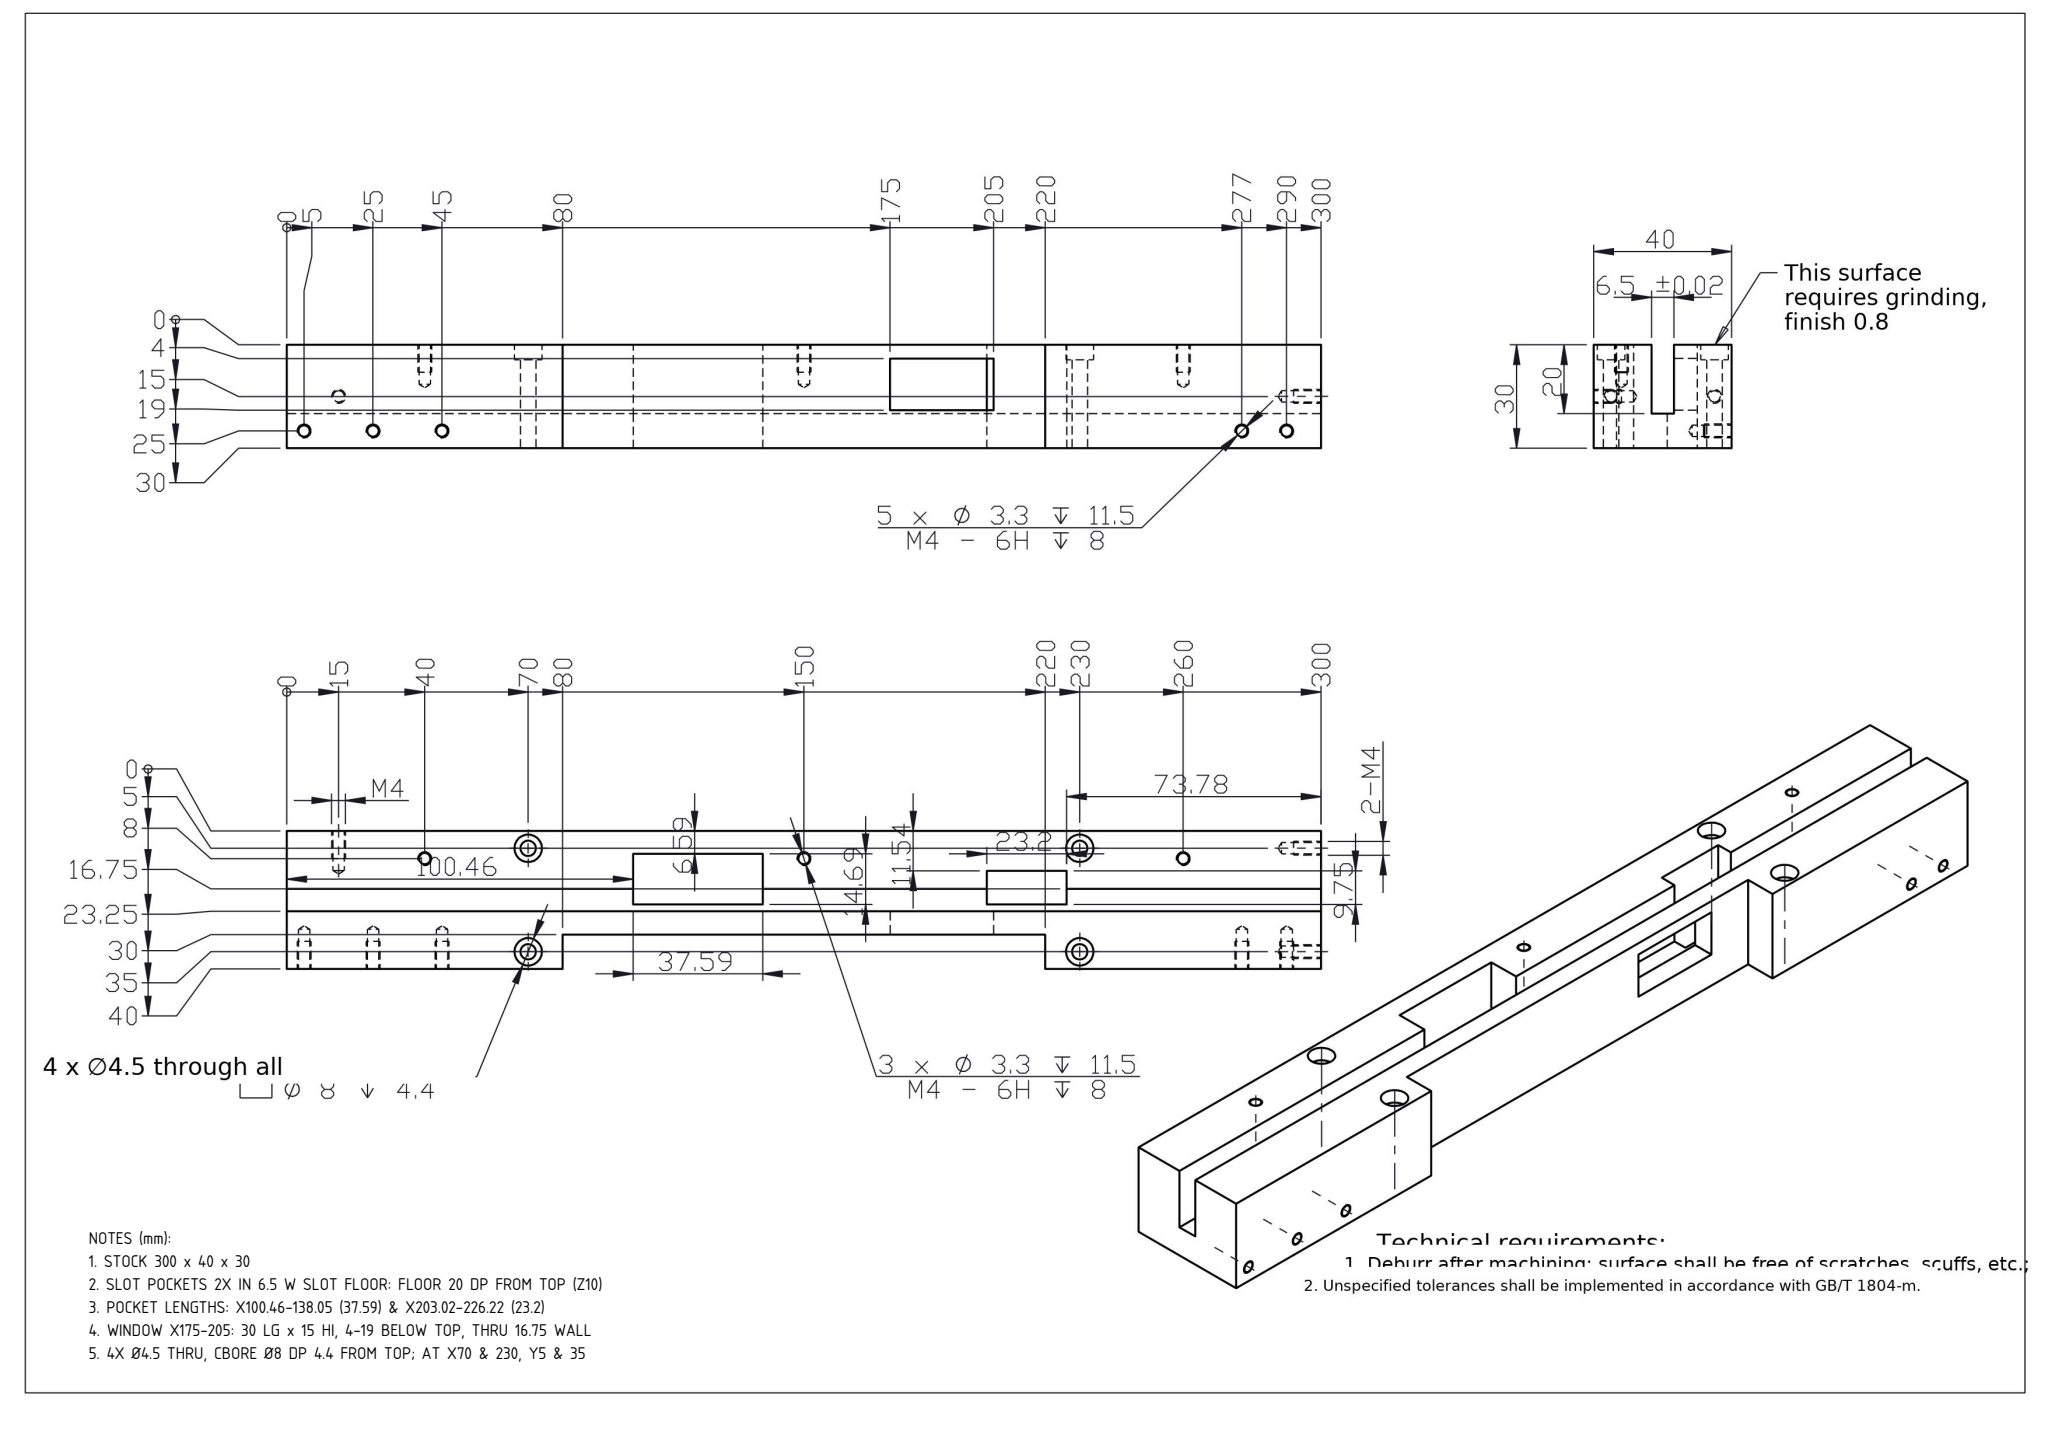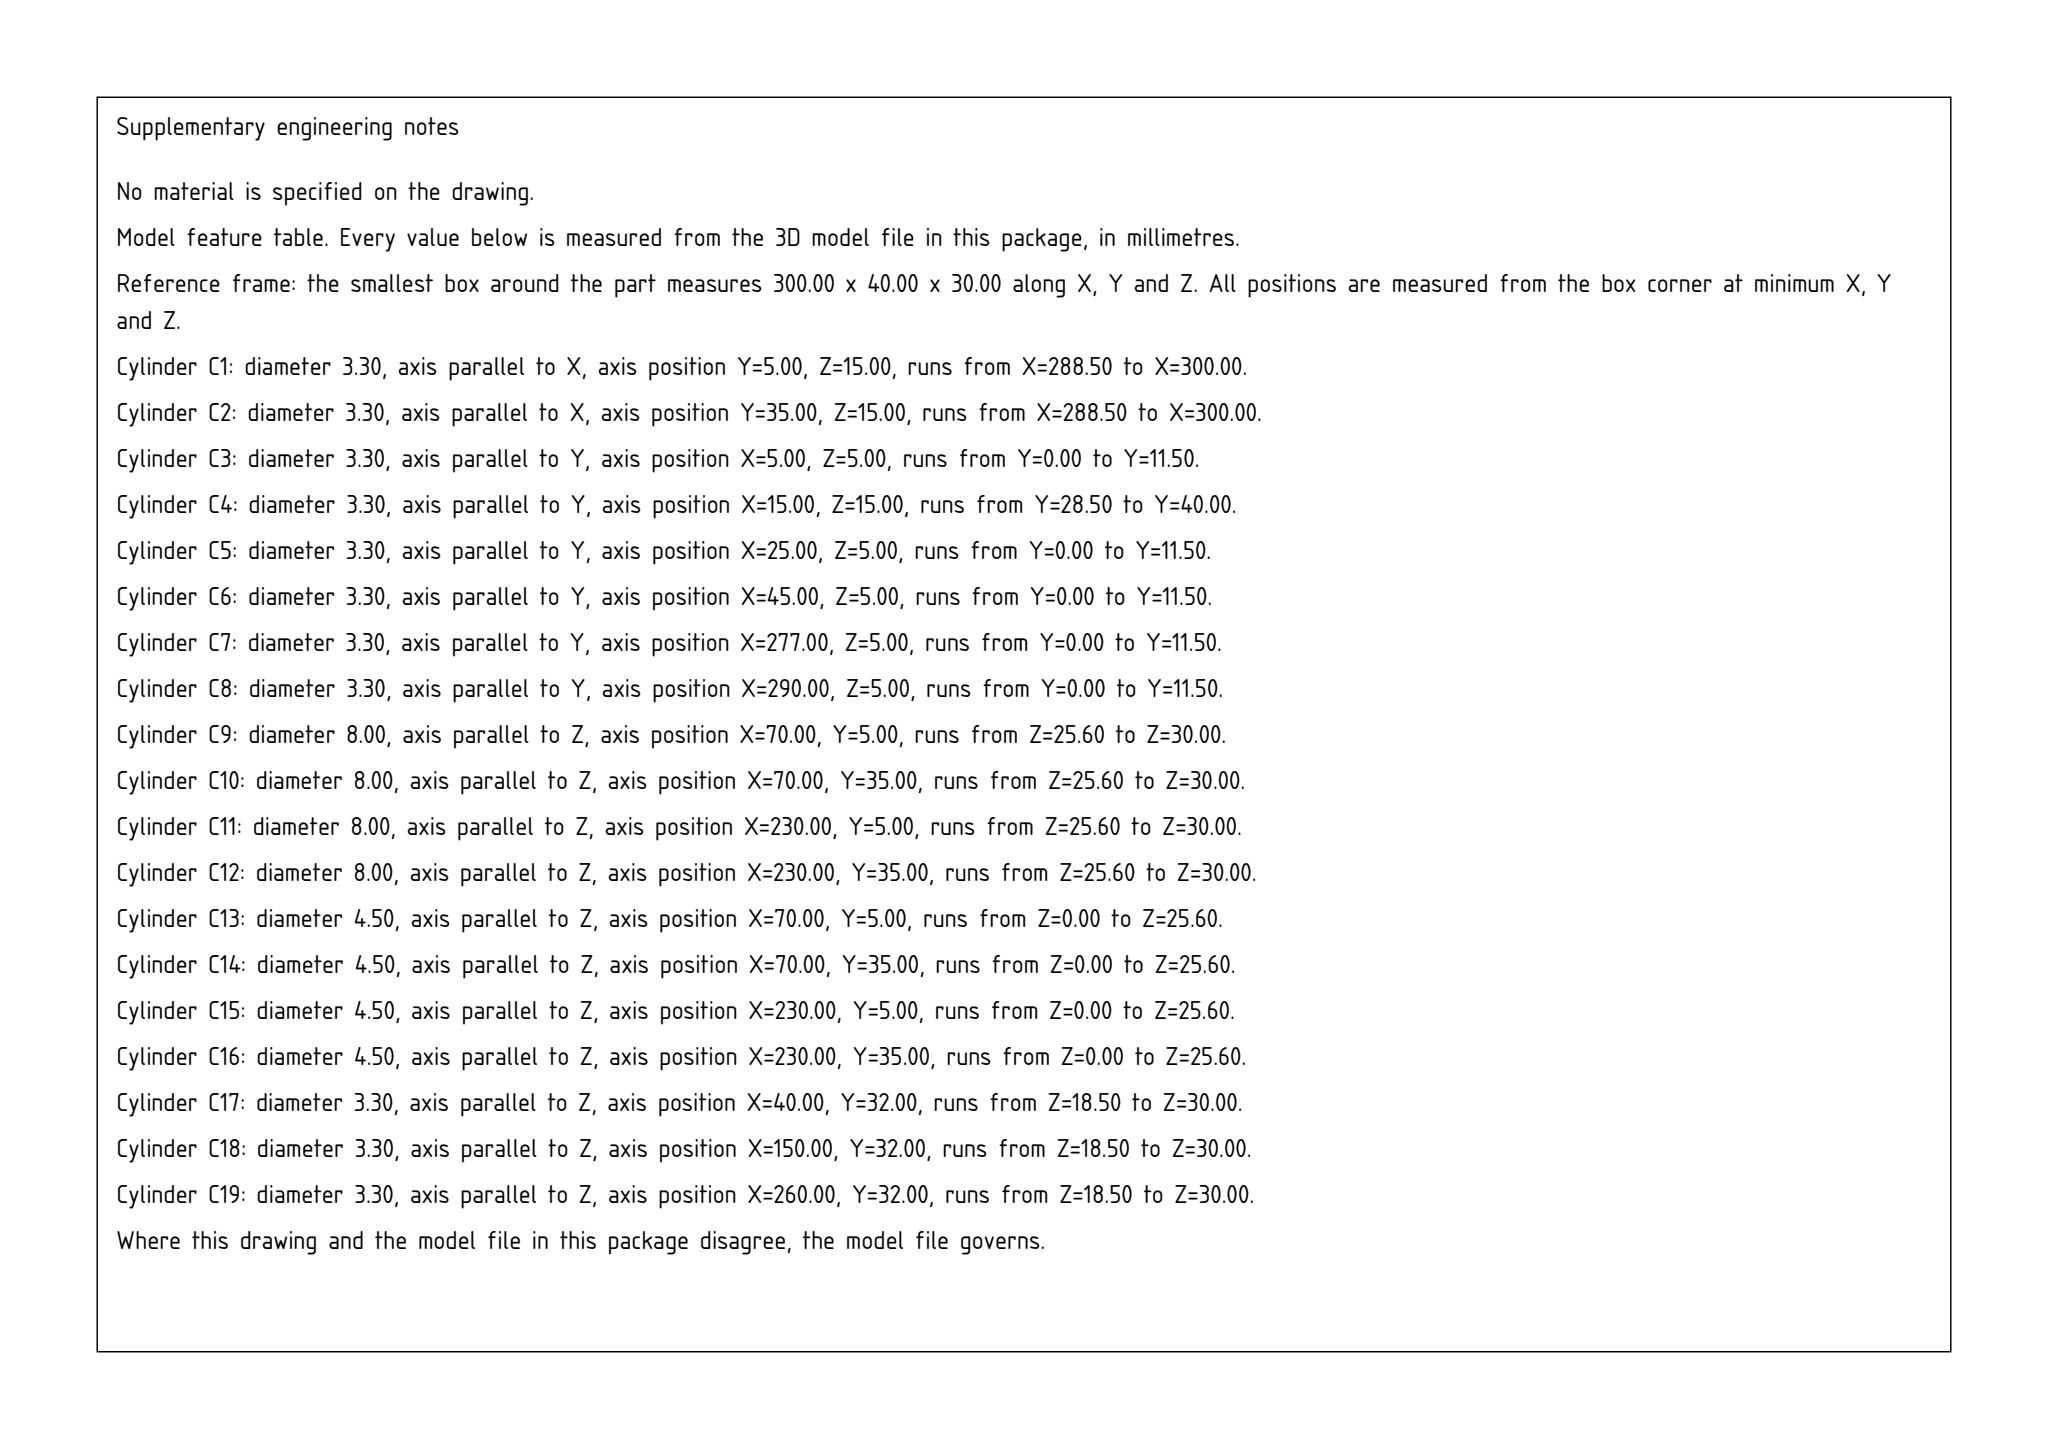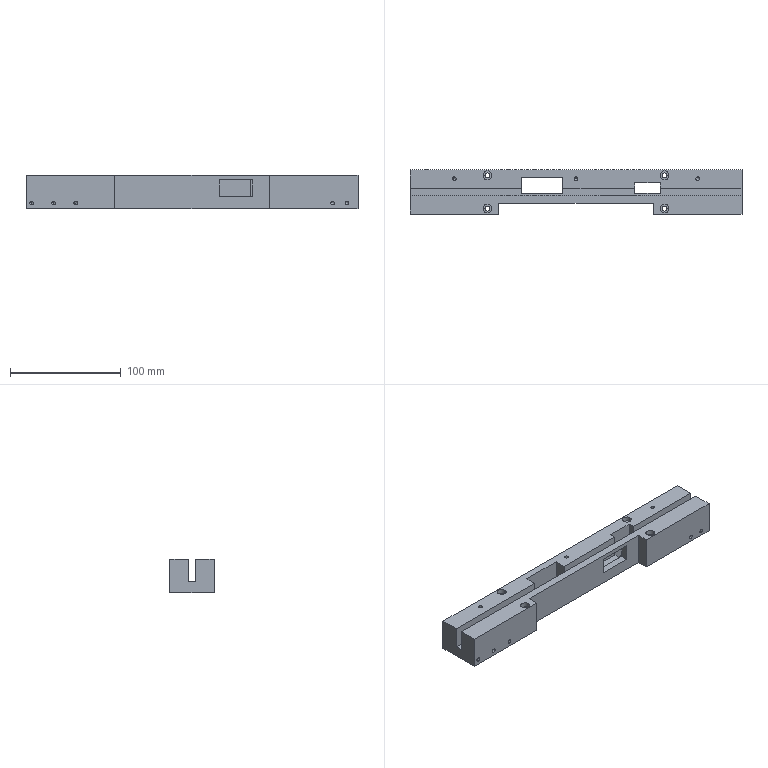Part | SolidWorks | mm | 1 solid | 92 faces | box 300 x 40 x 30 mm | volume 254494 mm3 | cylinder 38 | plane 32 | cone 22 | commonest cylinder face diameters 3.3 x22 8 x8 4.5 x8
Drawing notes:
STOCK 300 x 40 x 30 | from the solid: bbox_xyz 300.0 x 40.0 x 30.0
SLOT POCKETS 2X IN 6.5 W SLOT FLOOR: FLOOR 20 DP FROM TOP (Z10) | from the solid: y-planes 16.75 & 23.25 = 6.5 W; pocket floor z=10.0, 20 below z=30 top face
POCKET LENGTHS: X100.46-138.05 (37.59) & X203.02-226.22 (23.2) | from the solid: x-planes 100.46, 138.05, 203.02, 226.22
WINDOW X175-205: 30 LG x 15 HI, 4-19 BELOW TOP, THRU 16.75 WALL | from the solid: x-planes 175.0 & 205.0; z-planes 11.0 & 26.0; wall y=0 to y=16.75
4X Ø4.5 THRU, CBORE Ø8 DP 4.4 FROM TOP; AT X70 & 230, Y5 & 35 | from the solid: Ø4.5 axis z L25.6 and Ø8 axis z L4.4 at (70,5),(70,35),(230,5),(230,35); z-planes 25.6 & 30.0
build123d program:
from build123d import *

# Parameters (mm, degrees)
SKETCH1_W                                       = 300
SKETCH1_H                                       = 40
BOSS_EXTRUDE1_DEPTH                             = 30
SKETCH2_W                                       = 300
SKETCH2_H                                       = 6.5
CUT_EXTRUDE1_DEPTH                              = 20
M4_HEX_SOCKET_HEAD_CAP_SCREW_CBORE2_D           = 4.5
M4_HEX_SOCKET_HEAD_CAP_SCREW_CBORE2_CBORE_D     = 8
M4_HEX_SOCKET_HEAD_CAP_SCREW_CBORE2_CBORE_DEPTH = 4.4
M4_TAPPED_HOLE1_D                               = 3.3
M4_TAPPED_HOLE1_DEPTH                           = 11.5
M4_TAPPED_HOLE1_TIP                             = 0.9914
SKETCH13_W                                      = 140
SKETCH13_H                                      = 30
CUT_EXTRUDE2_DEPTH                              = 10
CUT_EXTRUDE3_REACH                              = 304.985
SKETCH14_W                                      = 30
SKETCH14_H                                      = 15
M4_TAPPED_HOLE2_D                               = 3.3
M4_TAPPED_HOLE2_DEPTH                           = 11.5
M4_TAPPED_HOLE2_TIP                             = 0.9914
M4_TAPPED_HOLE3_D                               = 3.3
M4_TAPPED_HOLE3_DEPTH                           = 11.5
M4_TAPPED_HOLE3_TIP                             = 0.9914
M4_TAPPED_HOLE4_D                               = 3.3
M4_TAPPED_HOLE4_DEPTH                           = 11.5
M4_TAPPED_HOLE4_TIP                             = 0.9914
M4_TAPPED_HOLE5_D                               = 3.3
M4_TAPPED_HOLE5_DEPTH                           = 11.5
M4_TAPPED_HOLE5_TIP                             = 0.9914
SKETCH23_W                                      = 23.203
SKETCH23_H                                      = 9.745
SKETCH23_W_2                                    = 37.588
SKETCH23_H_2                                    = 14.695
CUT_EXTRUDE4_DEPTH                              = 74


with BuildPart() as part:
    # Sketch1 → Boss-Extrude1 (new body)
    with BuildSketch(Plane.XY):
        with Locations((150, -20)):
            Rectangle(SKETCH1_W, SKETCH1_H)
    extrude(amount=BOSS_EXTRUDE1_DEPTH)

    # Sketch2 → Cut-Extrude1 (cut)
    with BuildSketch(Plane.XY.offset(30)):
        with Locations((150, -20)):
            Rectangle(SKETCH2_W, SKETCH2_H)
    extrude(amount=-CUT_EXTRUDE1_DEPTH, mode=Mode.SUBTRACT)

    # M4 Hex Socket Head Cap Screw CBORE2 (through all)
    with Locations(Plane.XY.offset(30)):
        with Locations((70, -35), (230, -35), (230, -5), (70, -5)):
            CounterBoreHole(M4_HEX_SOCKET_HEAD_CAP_SCREW_CBORE2_D / 2, M4_HEX_SOCKET_HEAD_CAP_SCREW_CBORE2_CBORE_D / 2, M4_HEX_SOCKET_HEAD_CAP_SCREW_CBORE2_CBORE_DEPTH)

    # M4 Tapped Hole1
    with Locations(Plane(origin=(0, -40, 0), x_dir=(-1, 0, 0), z_dir=(0, -1, 0))):
        with Locations((-25, -5), (-45, -5), (-5, -5)):
            Hole(M4_TAPPED_HOLE1_D / 2, depth=M4_TAPPED_HOLE1_DEPTH)
            with Locations((0, 0, -(M4_TAPPED_HOLE1_DEPTH + M4_TAPPED_HOLE1_TIP / 2))):  # 118° drill point
                Cone(0, M4_TAPPED_HOLE1_D / 2, M4_TAPPED_HOLE1_TIP, mode=Mode.SUBTRACT)

    # Sketch13 → Cut-Extrude2 (cut)
    with BuildSketch(Plane.XZ.offset(40)):
        with Locations((150, 15)):
            Rectangle(SKETCH13_W, SKETCH13_H)
    extrude(amount=-CUT_EXTRUDE2_DEPTH, mode=Mode.SUBTRACT)

    # Sketch14 → Cut-Extrude3 (cut, up to next)
    with BuildSketch(Plane.XZ.offset(30), mode=Mode.PRIVATE) as cut_extrude3_sk1:
        with Locations((190, 18.5)):
            Rectangle(SKETCH14_W, SKETCH14_H)
    cut_extrude3_tool1 = extrude(cut_extrude3_sk1.sketch, amount=-CUT_EXTRUDE3_REACH, mode=Mode.PRIVATE) & part.part
    add(cut_extrude3_tool1.solids().sort_by_distance((190, -30, 18.5))[0], mode=Mode.SUBTRACT)

    # M4 Tapped Hole2
    with Locations(Plane(origin=(0, -40, 0), x_dir=(-1, 0, 0), z_dir=(0, -1, 0))):
        with Locations((-290, -5), (-277, -5)):
            Hole(M4_TAPPED_HOLE2_D / 2, depth=M4_TAPPED_HOLE2_DEPTH)
            with Locations((0, 0, -(M4_TAPPED_HOLE2_DEPTH + M4_TAPPED_HOLE2_TIP / 2))):  # 118° drill point
                Cone(0, M4_TAPPED_HOLE2_D / 2, M4_TAPPED_HOLE2_TIP, mode=Mode.SUBTRACT)

    # M4 Tapped Hole3
    with Locations(Plane.XY.offset(30)):
        with Locations((40, -8), (260, -8), (150, -8)):
            Hole(M4_TAPPED_HOLE3_D / 2, depth=M4_TAPPED_HOLE3_DEPTH)
            with Locations((0, 0, -(M4_TAPPED_HOLE3_DEPTH + M4_TAPPED_HOLE3_TIP / 2))):  # 118° drill point
                Cone(0, M4_TAPPED_HOLE3_D / 2, M4_TAPPED_HOLE3_TIP, mode=Mode.SUBTRACT)

    # M4 Tapped Hole4
    with Locations(Plane(origin=(0, 0, 0), x_dir=(1, 0, 0), z_dir=(0, 1, 0))):
        with Locations((15, -15)):
            Hole(M4_TAPPED_HOLE4_D / 2, depth=M4_TAPPED_HOLE4_DEPTH)
            with Locations((0, 0, -(M4_TAPPED_HOLE4_DEPTH + M4_TAPPED_HOLE4_TIP / 2))):  # 118° drill point
                Cone(0, M4_TAPPED_HOLE4_D / 2, M4_TAPPED_HOLE4_TIP, mode=Mode.SUBTRACT)

    # M4 Tapped Hole5
    with Locations(Plane(origin=(300, 0, 0), x_dir=(0, 0, -1), z_dir=(1, 0, 0))):
        with Locations((-15, -35), (-15, -5)):
            Hole(M4_TAPPED_HOLE5_D / 2, depth=M4_TAPPED_HOLE5_DEPTH)
            with Locations((0, 0, -(M4_TAPPED_HOLE5_DEPTH + M4_TAPPED_HOLE5_TIP / 2))):  # 118° drill point
                Cone(0, M4_TAPPED_HOLE5_D / 2, M4_TAPPED_HOLE5_TIP, mode=Mode.SUBTRACT)

    # Sketch23 → Cut-Extrude4 (cut)
    with BuildSketch(Plane(origin=(0, 0, 0), x_dir=(-1, 0, 0), z_dir=(0, 0, -1))):
        with Locations((-214.619, -16.411)):
            Rectangle(SKETCH23_W, SKETCH23_H)
        with Locations((-119.256, -13.936)):
            Rectangle(SKETCH23_W_2, SKETCH23_H_2)
    extrude(amount=-CUT_EXTRUDE4_DEPTH, mode=Mode.SUBTRACT)


solid = part.part